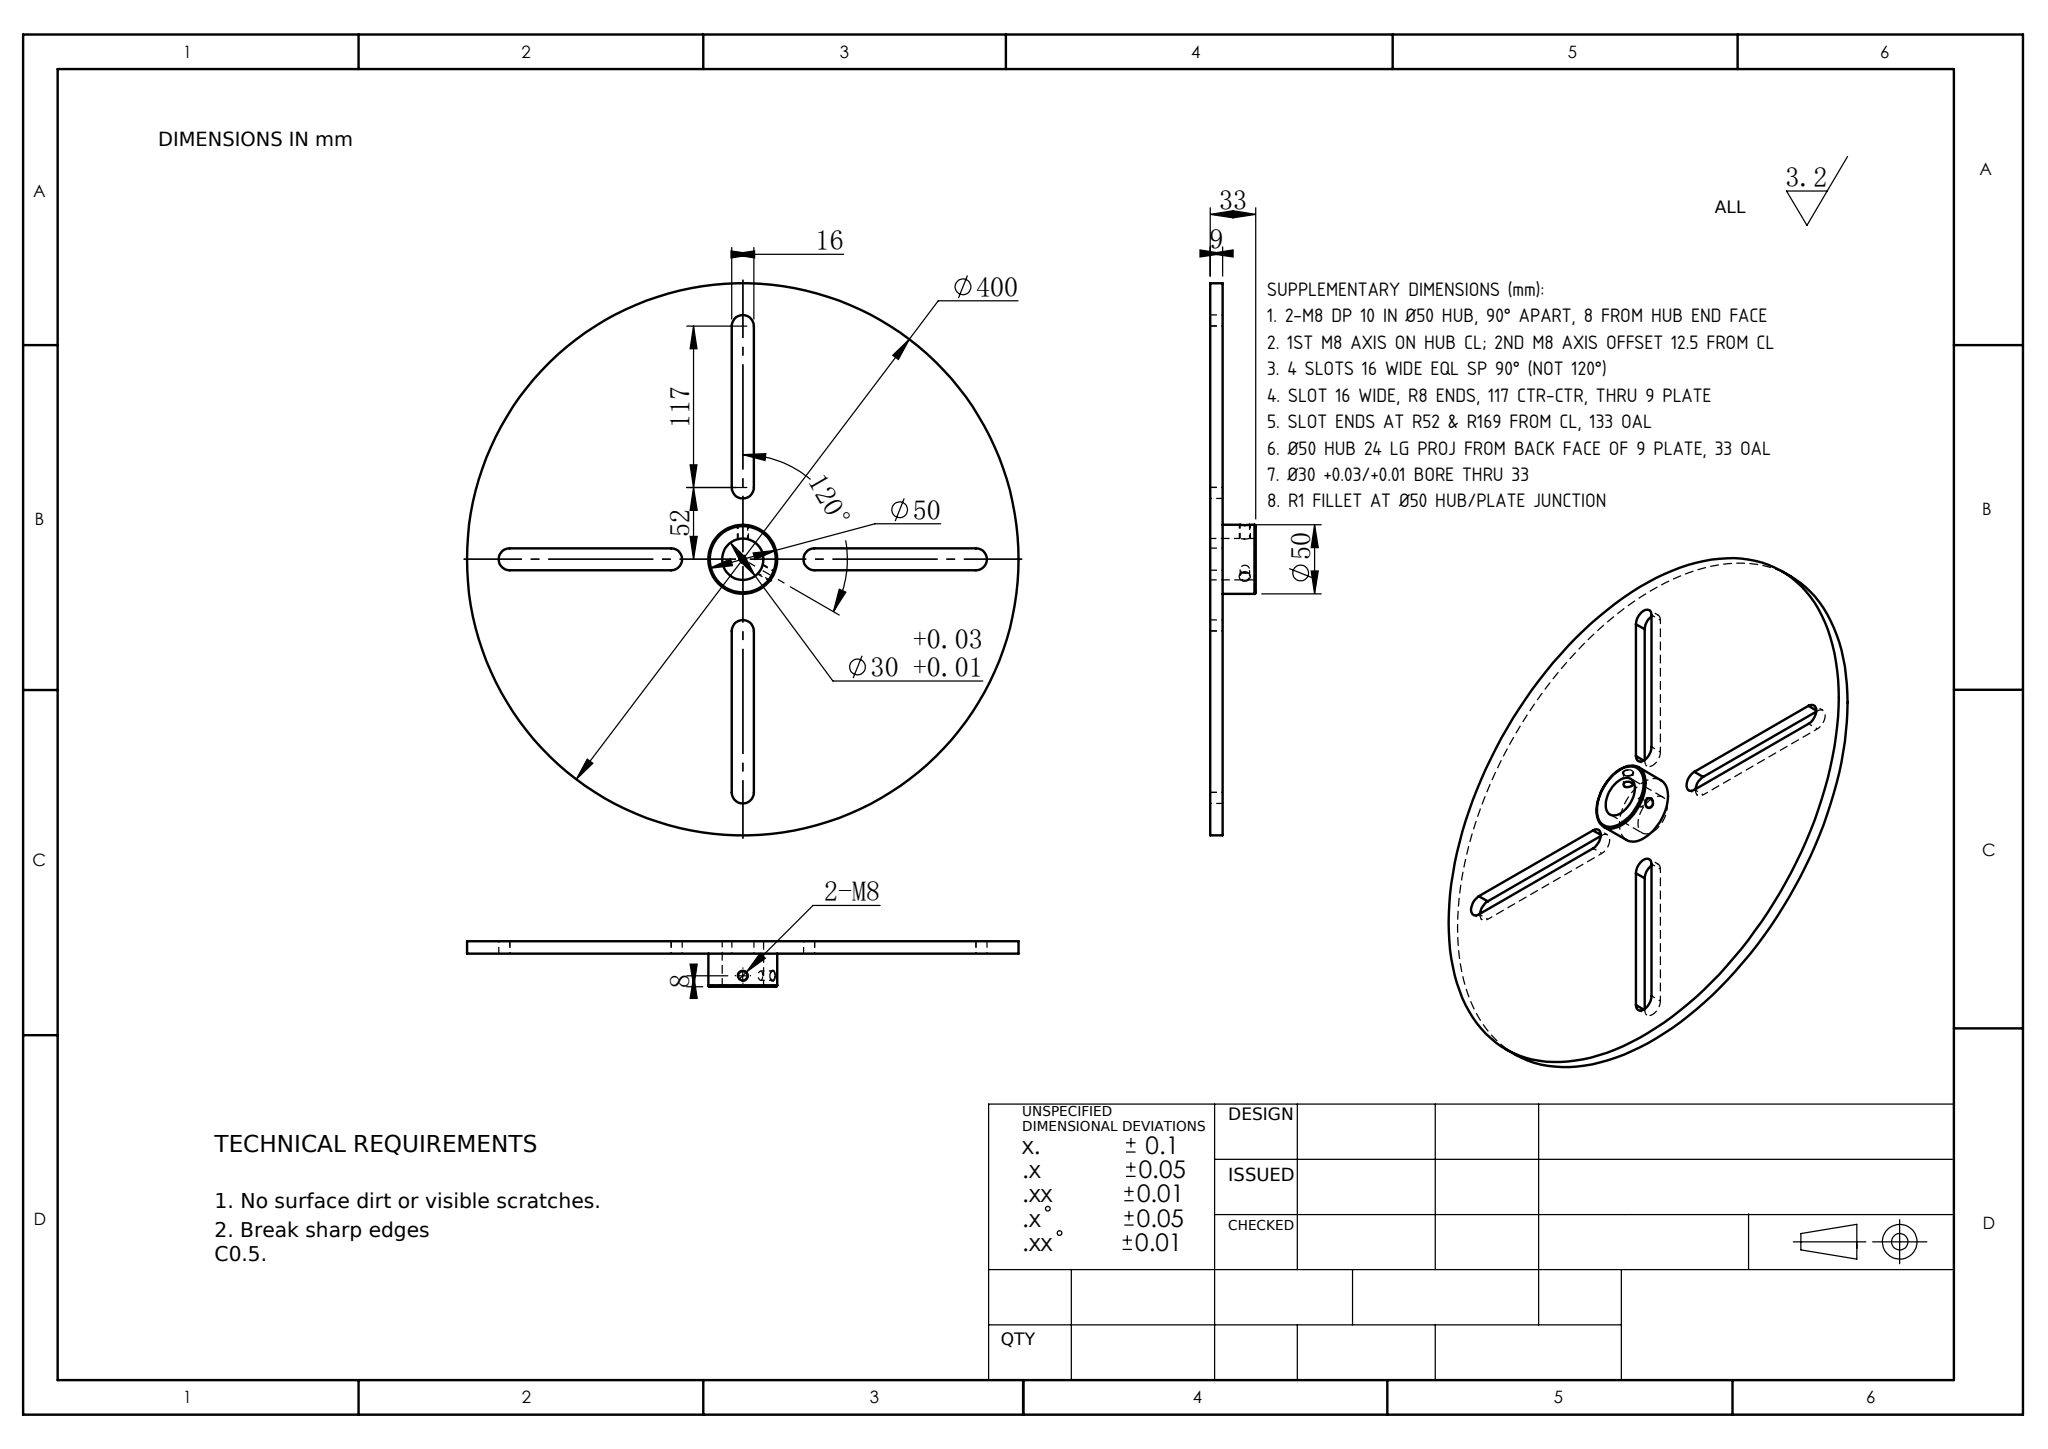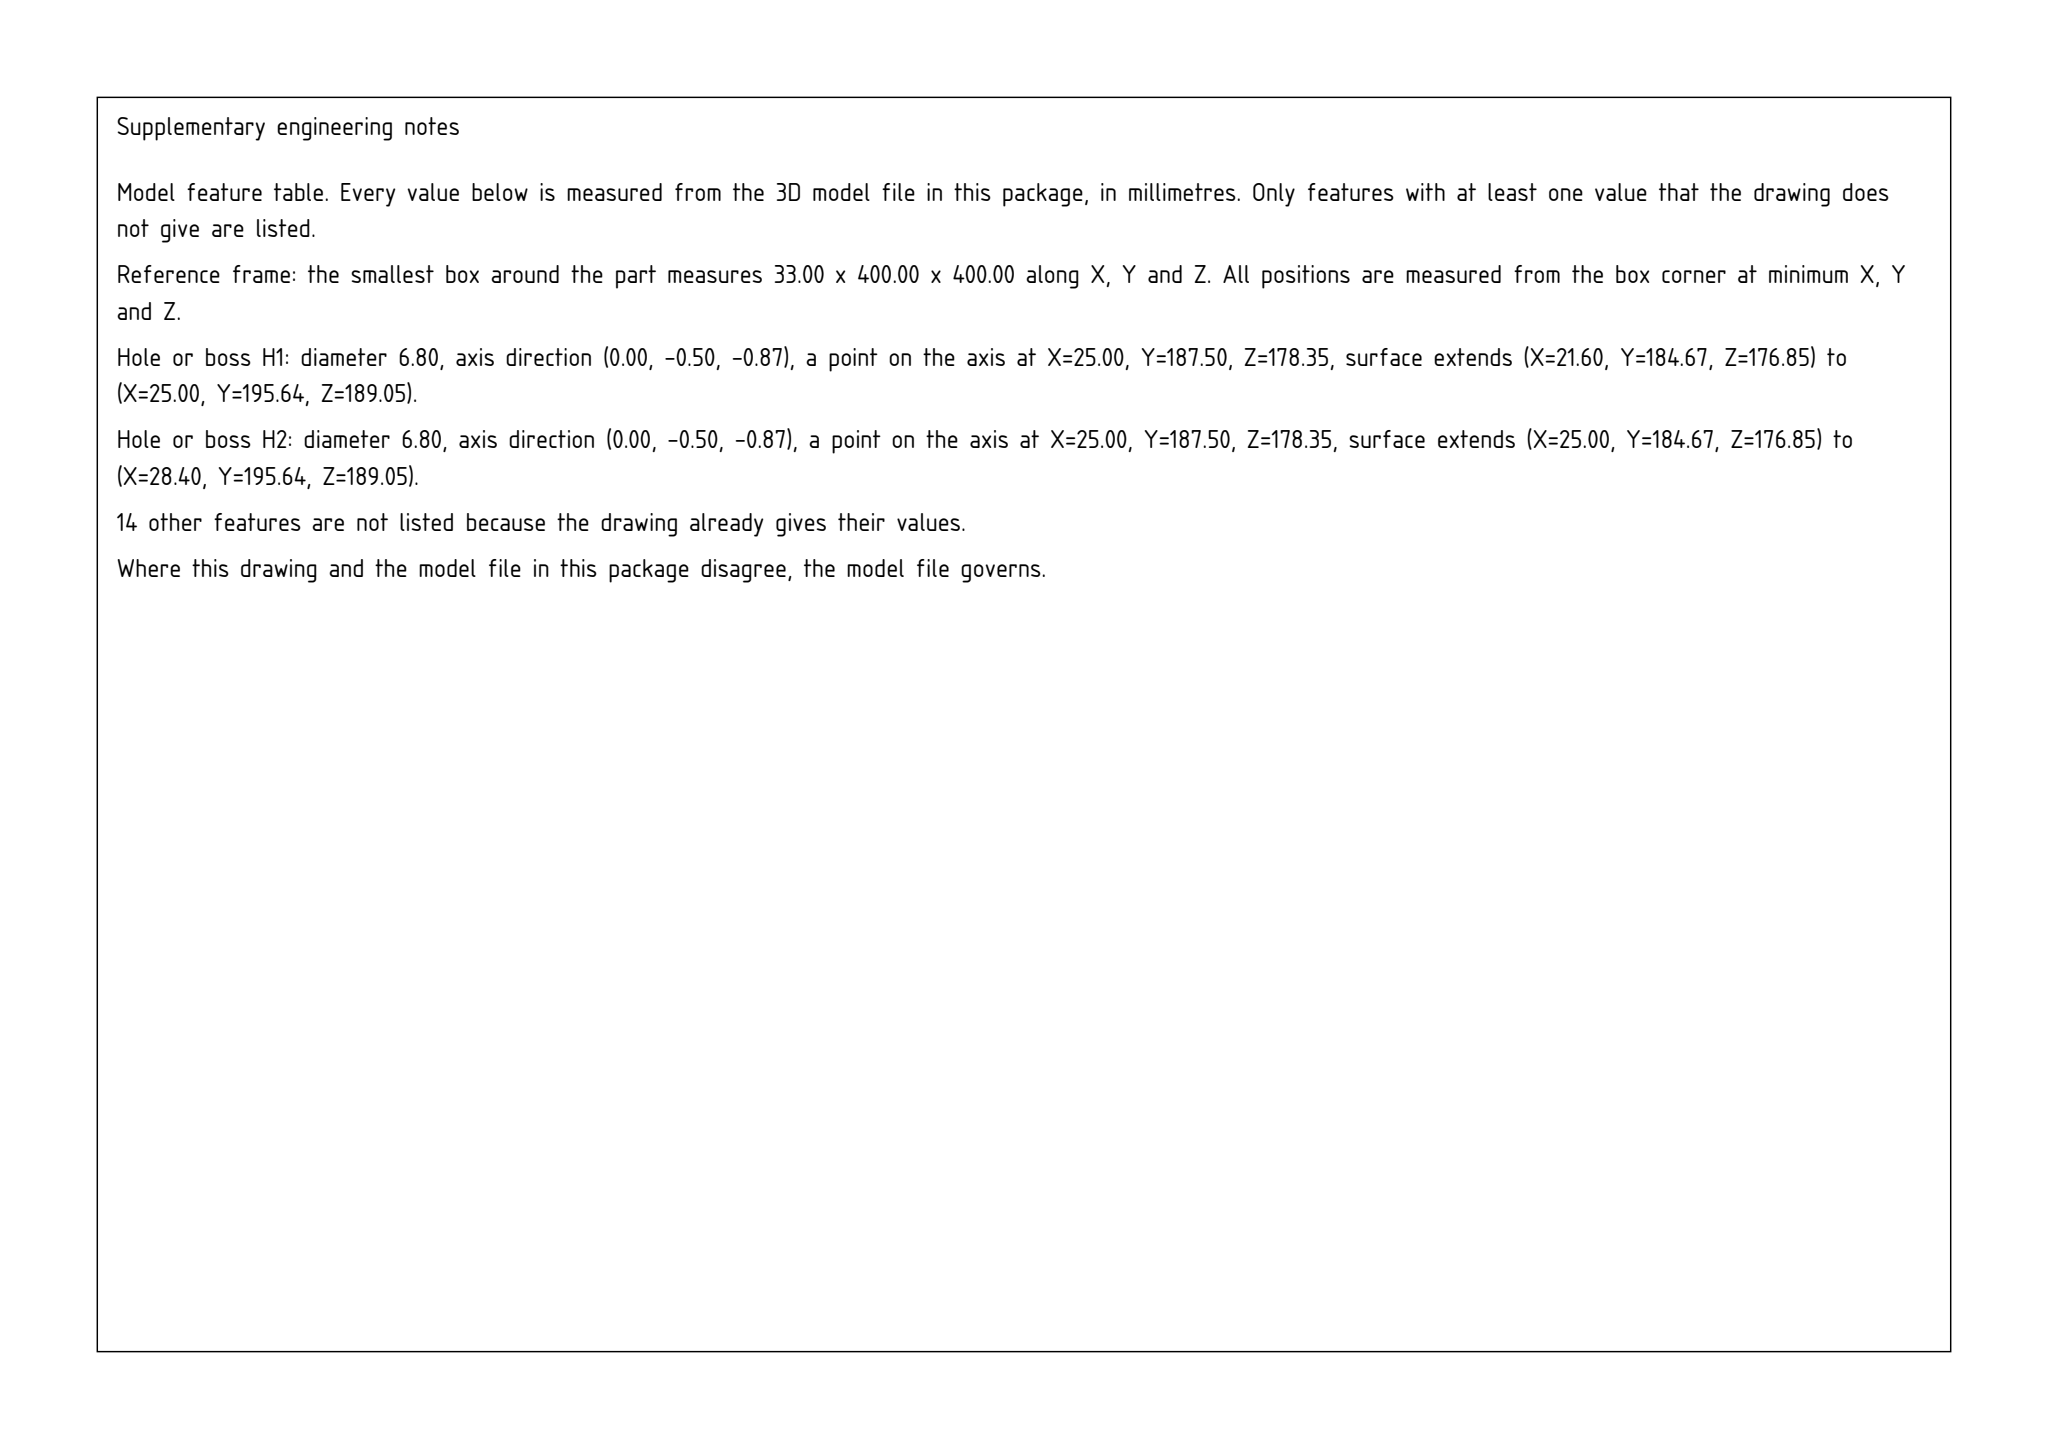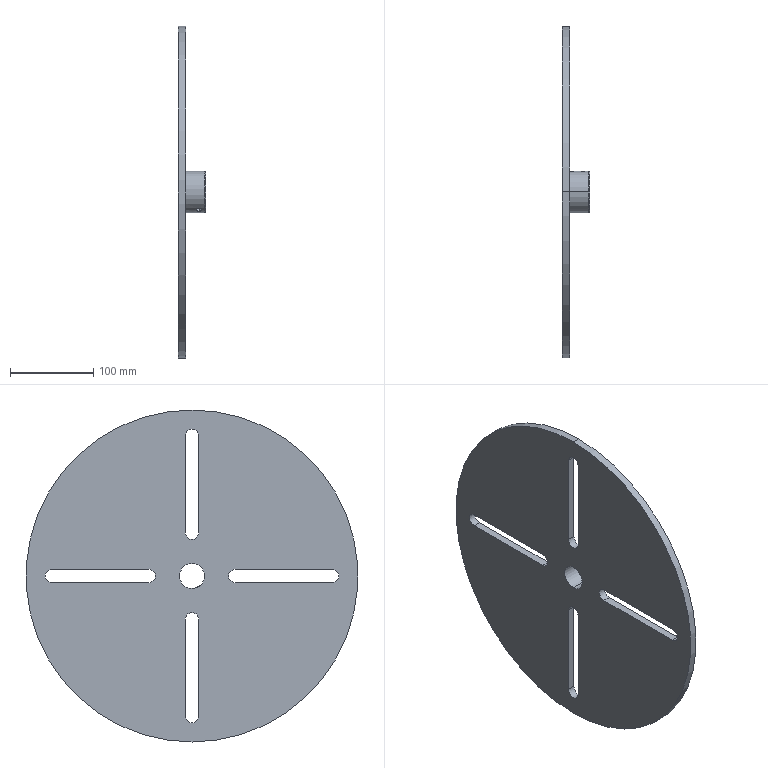Part | SolidWorks | mm | 1 solid | 33 faces | box 33 x 400 x 400 mm | volume 1079378 mm3 | cylinder 20 | plane 11 | torus 2 | commonest cylinder face diameters 16 x10 6.8 x4 50 x2 400 x2 30 x2
build123d program:
from build123d import *

# Parameters (mm, degrees)
CUT_EXTRUDE1_DEPTH     = 285.761
CIRPATTERN1_COUNT      = 4
FILLET1_R              = 1
M8_TAPPED_HOLE1_REACH  = 304.843
M8_TAPPED_HOLE1_BORE_R = 3.4
CIRPATTERN2_COUNT      = 2
CIRPATTERN2_ANGLE      = 120


with BuildPart() as part:
    # Sketch1 → Revolve1 (revolve)
    with BuildSketch(Plane.XY, mode=Mode.PRIVATE) as revolve1_sk:
        Polygon((0, 15), (0, 200), (9, 200), (9, 25), (33, 25), (33, 15), align=None)
    revolve(revolve1_sk.sketch.rotate(Axis((0, 0, 0), (-1, 0, 0)), 90), axis=Axis((0, 0, 0), (-1, 0, 0)))

    # Sketch2 → Cut-Extrude1 (cut, through all)
    with BuildSketch(Plane.ZY):
        with BuildLine():
            Line((8, -52), (8, -169))
            ThreePointArc((8, -169), (0, -177), (-8, -169))
            Line((-8, -169), (-8, -52))
            ThreePointArc((-8, -52), (0, -44), (8, -52))
        make_face()
    cut_extrude1 = extrude(amount=-CUT_EXTRUDE1_DEPTH, mode=Mode.SUBTRACT)

    # CirPattern1: Cut-Extrude1 ×4 about axis
    cirpattern1_axis = Axis((0, 0, 0), (1, 0, 0))
    for i in range(1, CIRPATTERN1_COUNT):
        add(cut_extrude1.rotate(cirpattern1_axis, i * 360 / CIRPATTERN1_COUNT), mode=Mode.SUBTRACT)

    # Fillet1
    fillet1_edges = [part.edges().sort_by_distance(p)[0] for p in [
        (33, 0, 25),
    ]]
    fillet(fillet1_edges, radius=FILLET1_R)

    # M8 Tapped Hole1 bore → M8 Tapped Hole1 (cut, up to next)
    with BuildSketch(Plane(origin=(0, 25, 0), x_dir=(1, 0, 0), z_dir=(0, 1, 0)), mode=Mode.PRIVATE) as m8_tapped_hole1_sk1:
        with Locations((25, 0)):
            Circle(M8_TAPPED_HOLE1_BORE_R)
    m8_tapped_hole1_tool1 = extrude(m8_tapped_hole1_sk1.sketch, amount=-M8_TAPPED_HOLE1_REACH, mode=Mode.PRIVATE) & part.part
    m8_tapped_hole1 = m8_tapped_hole1_tool1.solids().sort_by_distance((25, 25, 0))[0]
    add(m8_tapped_hole1, mode=Mode.SUBTRACT)

    # CirPattern2: M8 Tapped Hole1 ×2 about axis
    cirpattern2_axis = Axis((33, 0, 0), (-1, 0, 0))
    for i in range(1, CIRPATTERN2_COUNT):
        add(m8_tapped_hole1.rotate(cirpattern2_axis, i * CIRPATTERN2_ANGLE / (CIRPATTERN2_COUNT - 1)), mode=Mode.SUBTRACT)


solid = part.part